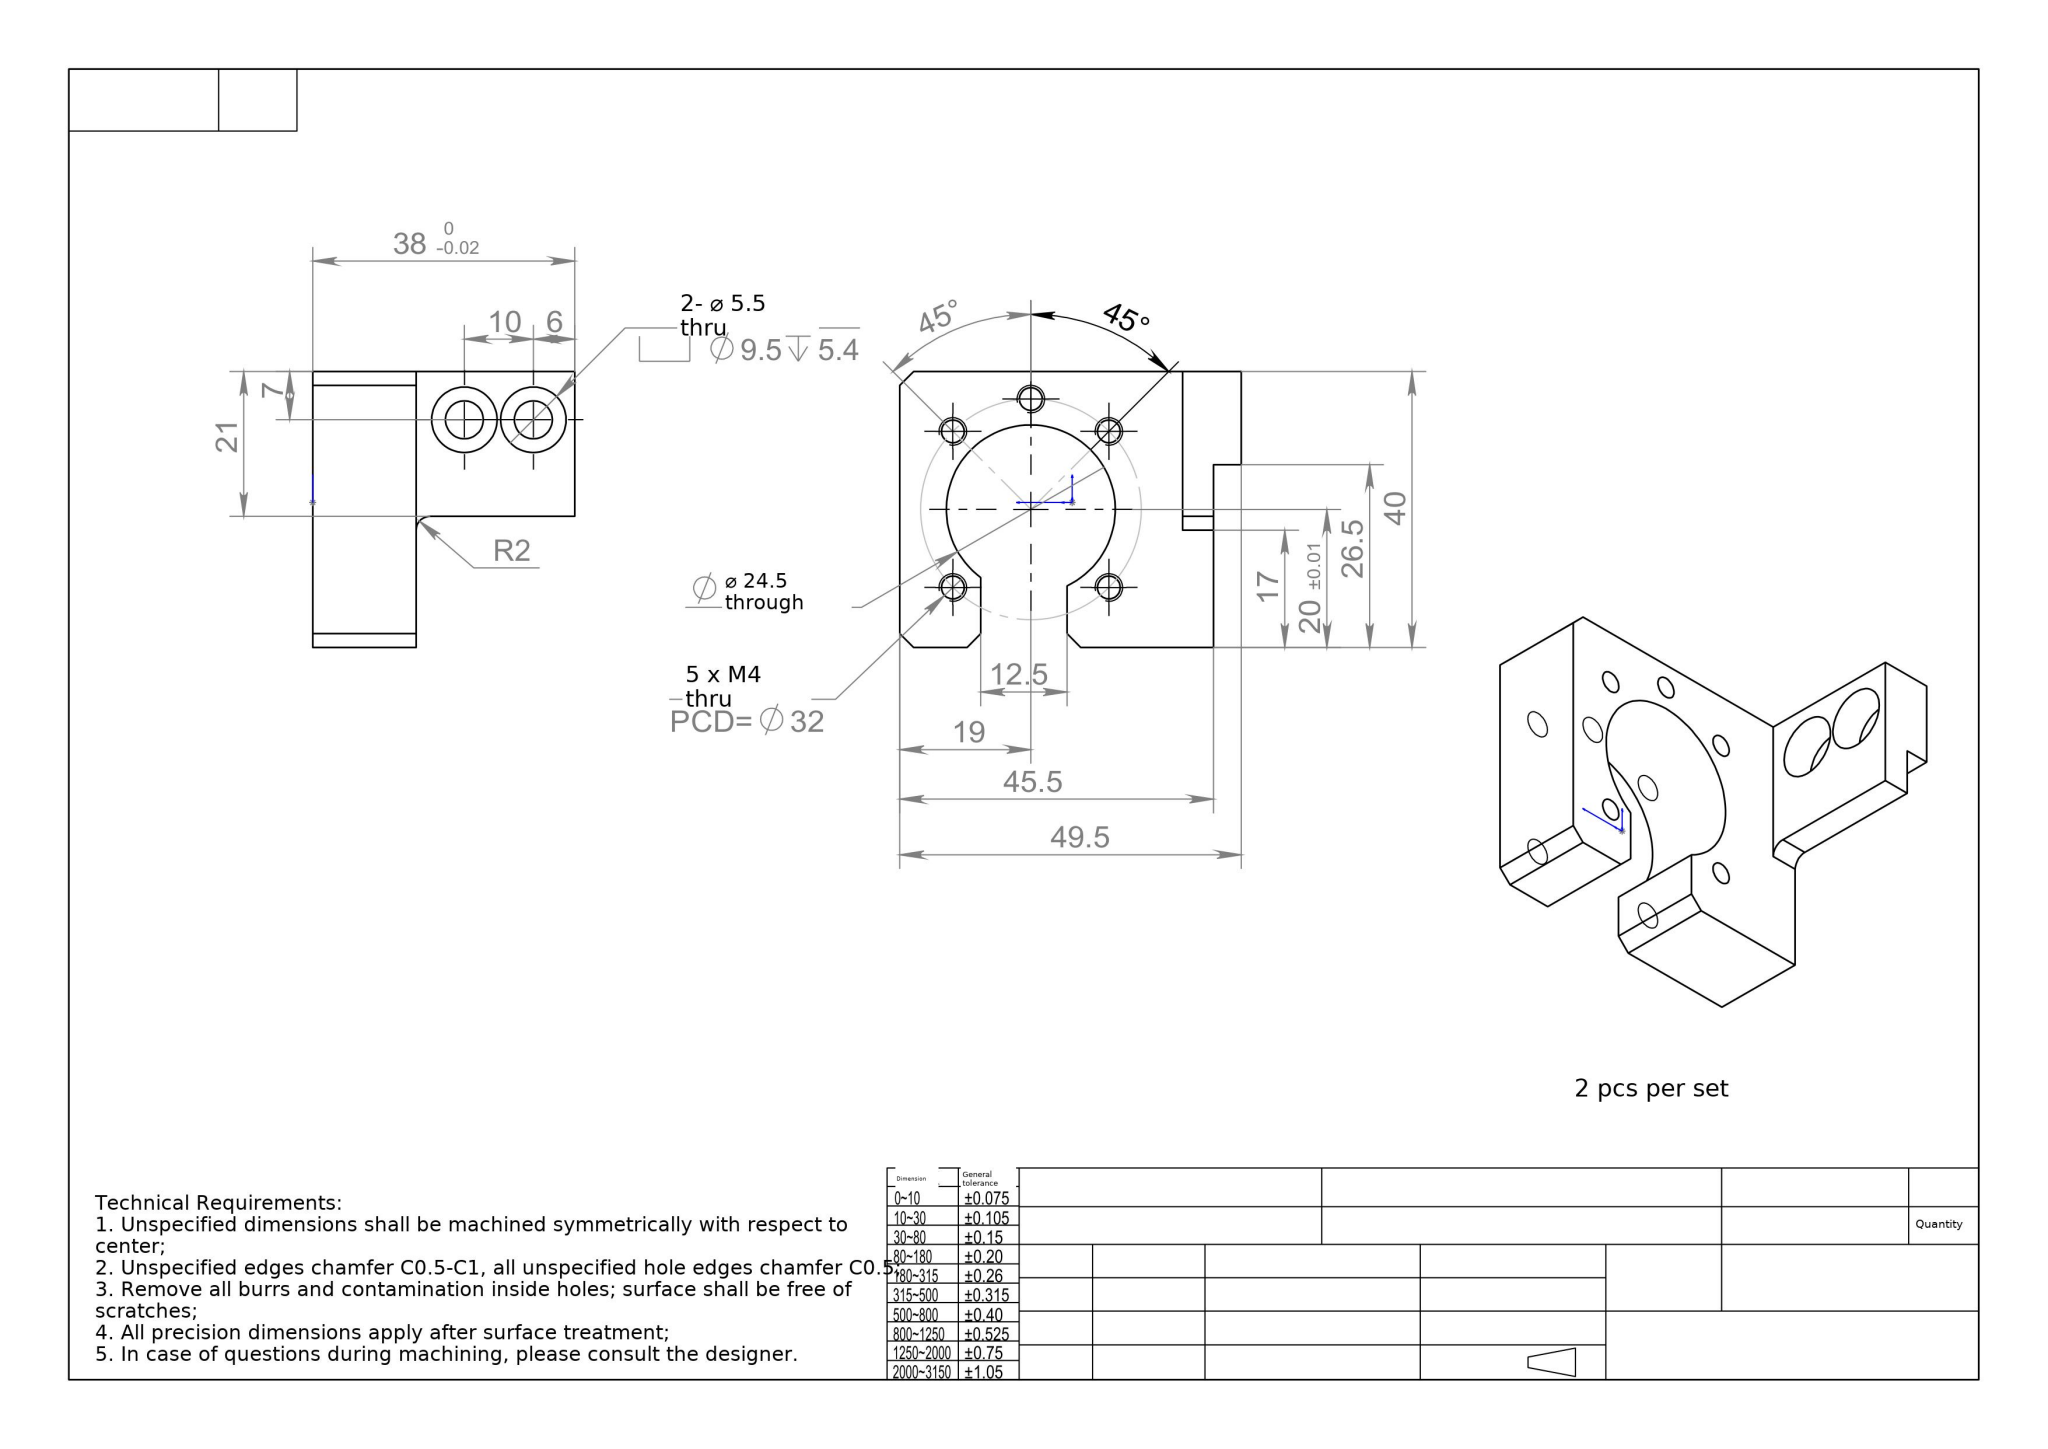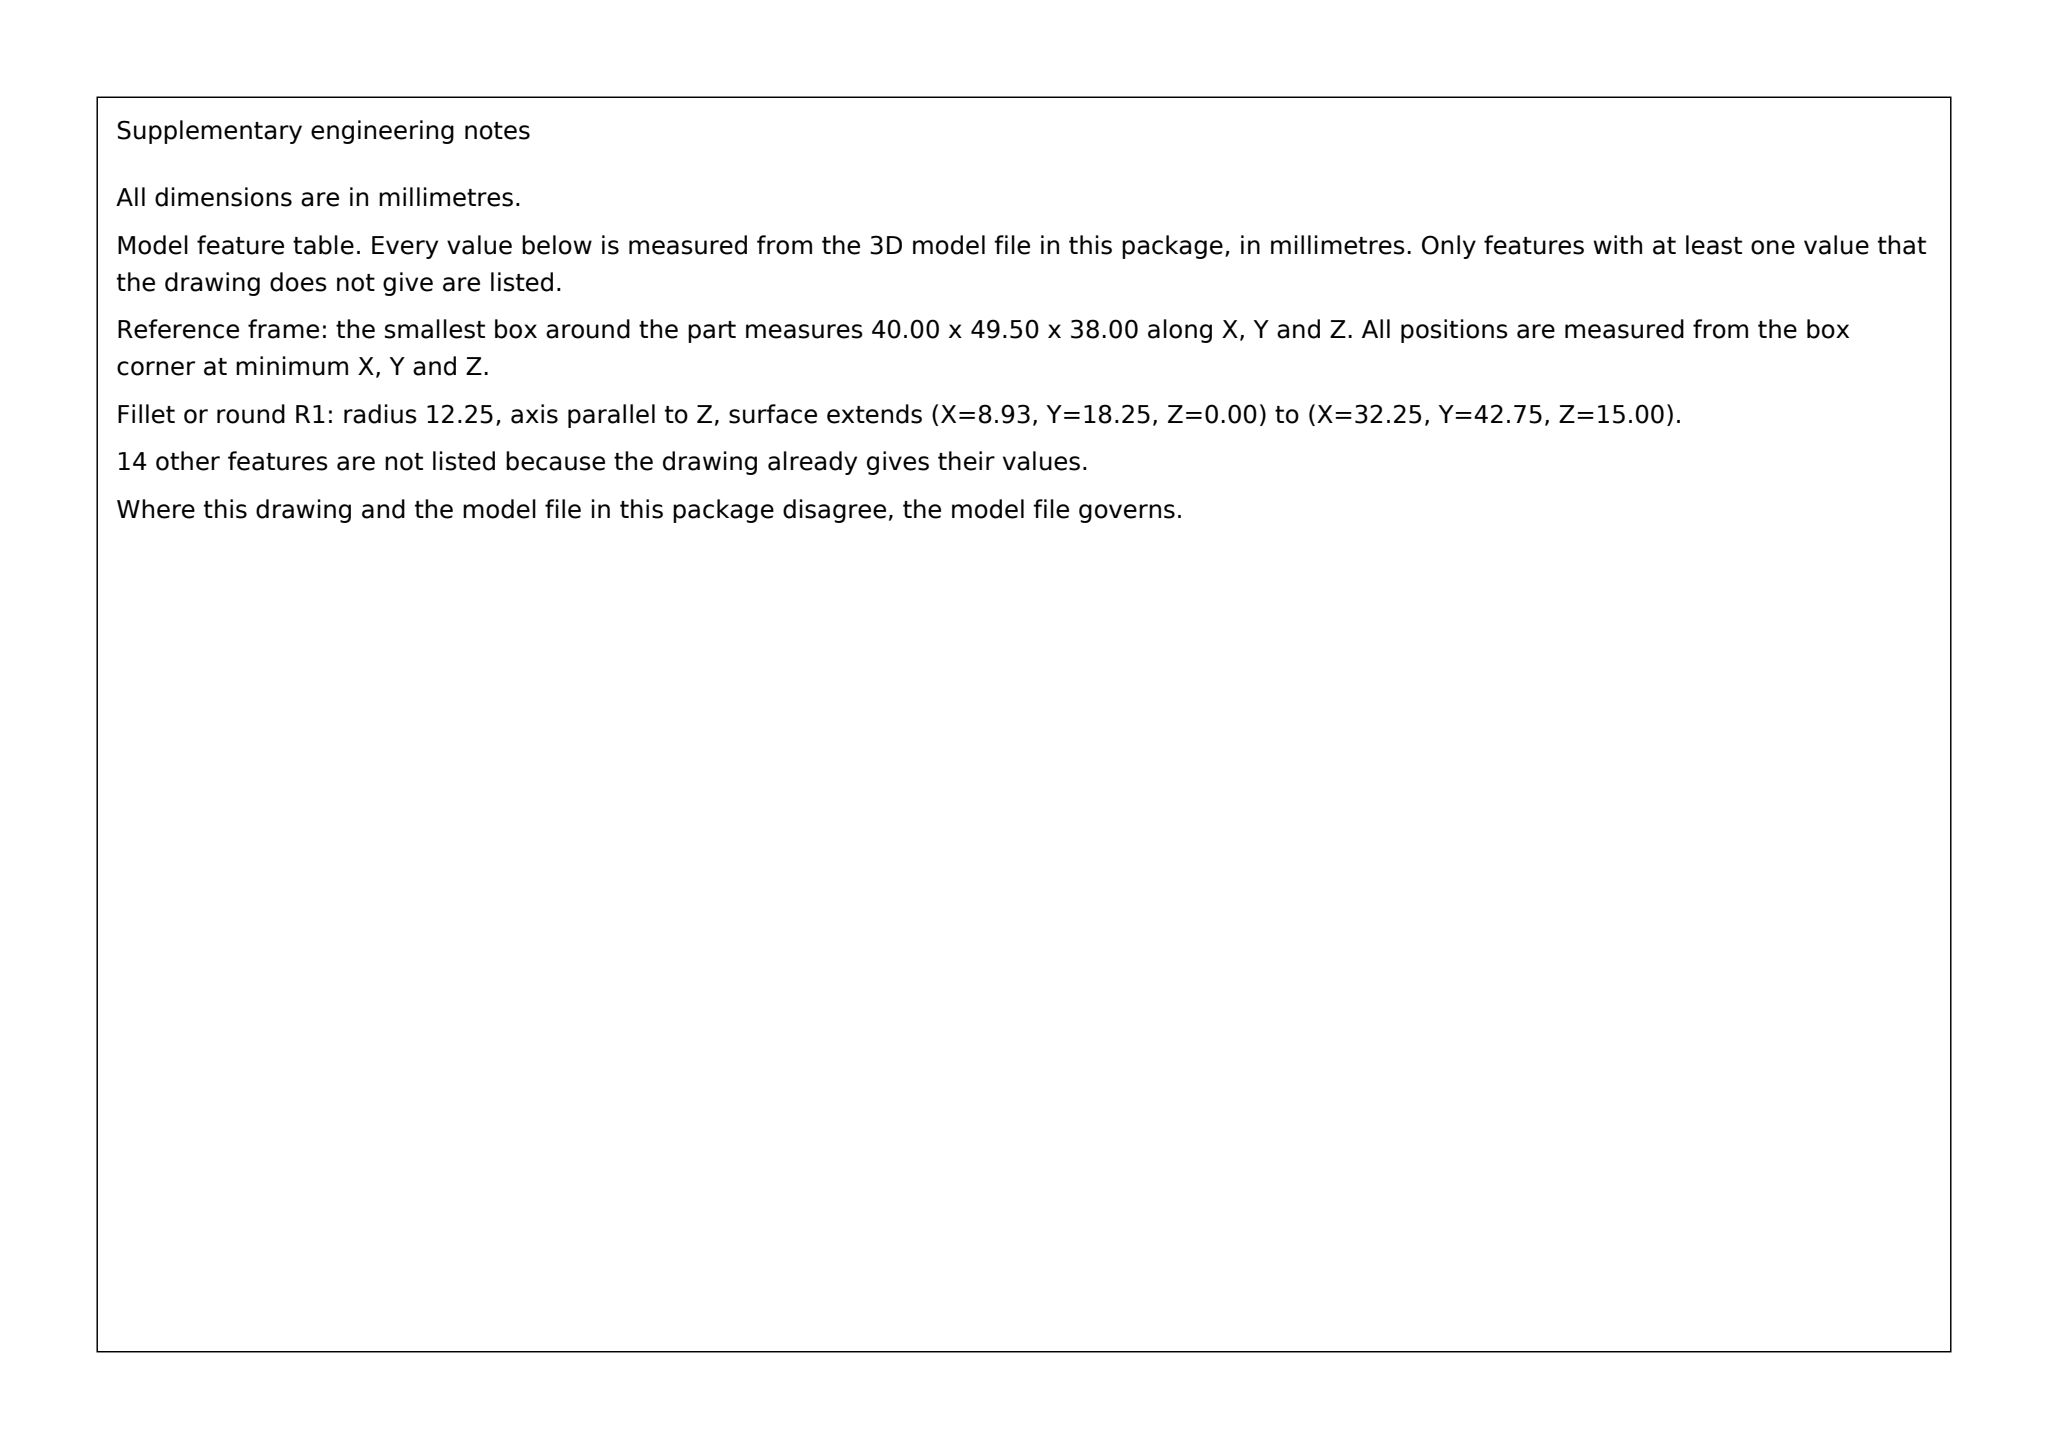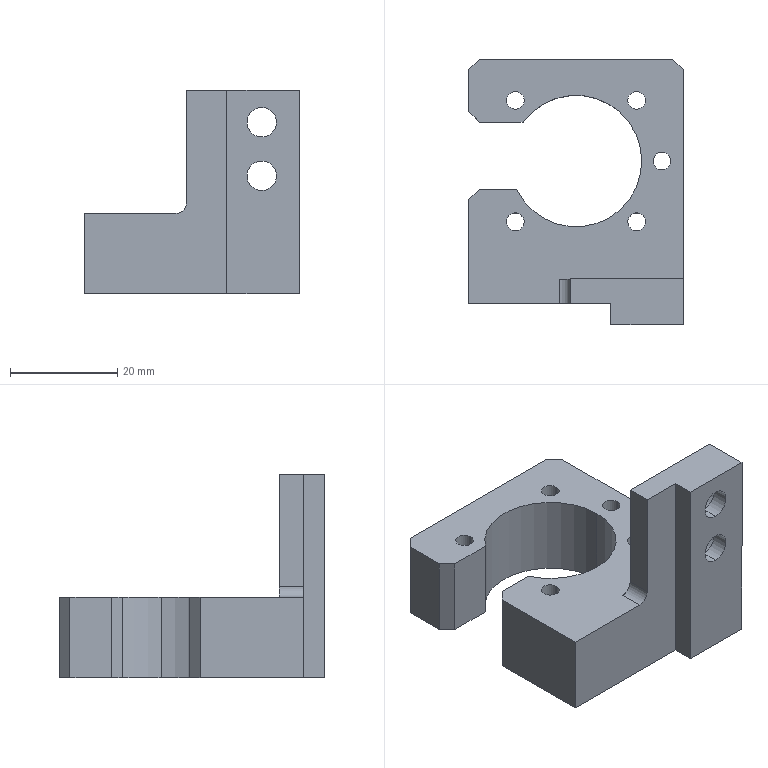Part | SolidWorks | mm | 1 solid | 41 faces | box 40 x 49.5 x 38 mm | volume 21218 mm3 | cylinder 21 | plane 20 | commonest cylinder face diameters 3.3 x10 9.5 x4 5.5 x4 24.5 x2 4 x1
build123d program:
from build123d import *

# Parameters (mm, degrees)
SKETCH1_W                                       = 42
SKETCH1_H                                       = 50
BOSS_EXTRUDE1_DEPTH                             = 15
SKETCH2_W                                       = 23
SKETCH2_H                                       = 9
BOSS_EXTRUDE2_DEPTH                             = 23
FILLET1_R                                       = 2
M5_HEX_SOCKET_HEAD_CAP_SCREW_CBORE1_D           = 5.5
M5_HEX_SOCKET_HEAD_CAP_SCREW_CBORE1_CBORE_D     = 9.5
M5_HEX_SOCKET_HEAD_CAP_SCREW_CBORE1_CBORE_DEPTH = 5.4
SKETCH5_R                                       = 12.25
CUT_EXTRUDE1_DEPTH                              = 40.937
SKETCH6_W                                       = 15
SKETCH6_H                                       = 12.5
CUT_EXTRUDE2_DEPTH                              = 40.937
SKETCH8_W                                       = 30
SKETCH8_H                                       = 0.5
CUT_EXTRUDE4_DEPTH                              = 51.1
CHAMFER2_SIZE                                   = 2
BOSS_EXTRUDE3_START                             = 2
SKETCH12_R                                      = 2.75
BOSS_EXTRUDE3_DEPTH                             = 2
M4_TAPPED_HOLE1_D                               = 3.3
SKETCH24_W                                      = 12
SKETCH24_H                                      = 38
CUT_EXTRUDE5_DEPTH                              = 2.5
M5_HEX_SOCKET_HEAD_CAP_SCREW_CBORE2_D           = 5.5
M5_HEX_SOCKET_HEAD_CAP_SCREW_CBORE2_CBORE_D     = 9.5
M5_HEX_SOCKET_HEAD_CAP_SCREW_CBORE2_CBORE_DEPTH = 5.4
SKETCH27_W                                      = 26.5
SKETCH27_H                                      = 4
CUT_EXTRUDE6_DEPTH                              = 51.1
SKETCH28_W                                      = 2
SKETCH28_H                                      = 38
CUT_EXTRUDE7_DEPTH                              = 66.843
CHAMFER3_SIZE                                   = 2


with BuildPart() as part:
    # Sketch1 → Boss-Extrude1 (new body)
    with BuildSketch(Plane.XY):
        Rectangle(SKETCH1_W, SKETCH1_H)
    extrude(amount=BOSS_EXTRUDE1_DEPTH)

    # Sketch2 → Boss-Extrude2 (add)
    with BuildSketch(Plane.XY.offset(15)):
        with Locations((9.5, -20.5)):
            Rectangle(SKETCH2_W, SKETCH2_H)
    extrude(amount=BOSS_EXTRUDE2_DEPTH)

    # Fillet1
    fillet1_edges = [part.edges().sort_by_distance(p)[0] for p in [
        (-2, -20.5, 15),
    ]]
    fillet(fillet1_edges, radius=FILLET1_R)

    # M5 Hex Socket Head Cap Screw CBORE1 (through all)
    with Locations(Plane(origin=(0, -16, 0), x_dir=(1, 0, 0), z_dir=(0, 1, 0))):
        with Locations((12, -32)):
            CounterBoreHole(M5_HEX_SOCKET_HEAD_CAP_SCREW_CBORE1_D / 2, M5_HEX_SOCKET_HEAD_CAP_SCREW_CBORE1_CBORE_D / 2, M5_HEX_SOCKET_HEAD_CAP_SCREW_CBORE1_CBORE_DEPTH)

    # Sketch5 → Cut-Extrude1 (cut, through all)
    with BuildSketch(Plane.XY.offset(15)):
        with Locations((-1, 6)):
            Circle(SKETCH5_R)
    extrude(amount=-CUT_EXTRUDE1_DEPTH, mode=Mode.SUBTRACT)

    # Sketch6 → Cut-Extrude2 (cut, through all)
    with BuildSketch(Plane.XY.offset(15)):
        with Locations((-13.5, 7)):
            Rectangle(SKETCH6_W, SKETCH6_H)
    extrude(amount=-CUT_EXTRUDE2_DEPTH, mode=Mode.SUBTRACT)

    # Sketch8 → Cut-Extrude4 (cut, through all)
    with BuildSketch(Plane(origin=(0, 0, 0), x_dir=(-1, 0, 0), z_dir=(0, 0, -1))):
        with Locations((6, -24.75)):
            Rectangle(SKETCH8_W, SKETCH8_H)
    extrude(amount=-CUT_EXTRUDE4_DEPTH, mode=Mode.SUBTRACT)

    # Chamfer2
    chamfer2_edges = [part.edges().sort_by_distance(p)[0] for p in [
        (-21, 13.25, 7.5),
        (-21, 0.75, 7.5),
        (-21, -24.5, 7.5),
        (-21, 25, 7.5),
    ]]
    chamfer(chamfer2_edges, length=CHAMFER2_SIZE)

    # Sketch12 → Boss-Extrude3 (add)
    with BuildSketch(Plane.XZ.offset(25).offset(BOSS_EXTRUDE3_START)):
        Polygon((9, 0), (21, 0), (21, 32), (21, 38), (9, 38), align=None)
        with Locations(Location((12, 32, 0), (0, 0, 90))):
            Circle(SKETCH12_R, mode=Mode.SUBTRACT)
        with Locations(Location((14.75, 21.349, 0), (0, 0, 270))):
            Circle(SKETCH12_R, mode=Mode.SUBTRACT)
    extrude(amount=-BOSS_EXTRUDE3_DEPTH)

    # M4 Tapped Hole1 (through all)
    with Locations(Plane(origin=(0, 0, 0), x_dir=(-1, 0, 0), z_dir=(0, 0, -1))):
        with Locations((-15, 6), (-10.314, 17.314), (-10.314, -5.314), (12.314, -5.314), (12.314, 17.314)):
            Hole(M4_TAPPED_HOLE1_D / 2)

    # Sketch24 → Cut-Extrude5 (cut)
    with BuildSketch(Plane.XZ.offset(27)):
        with Locations((15, 19)):
            Rectangle(SKETCH24_W, SKETCH24_H)
    extrude(amount=-CUT_EXTRUDE5_DEPTH, mode=Mode.SUBTRACT)

    # M5 Hex Socket Head Cap Screw CBORE2 (through all)
    with Locations(Plane(origin=(0, -16, 0), x_dir=(1, 0, 0), z_dir=(0, 1, 0))):
        with Locations((12, -22)):
            CounterBoreHole(M5_HEX_SOCKET_HEAD_CAP_SCREW_CBORE2_D / 2, M5_HEX_SOCKET_HEAD_CAP_SCREW_CBORE2_CBORE_D / 2, M5_HEX_SOCKET_HEAD_CAP_SCREW_CBORE2_CBORE_DEPTH)

    # Sketch27 → Cut-Extrude6 (cut, through all)
    with BuildSketch(Plane(origin=(0, 0, 0), x_dir=(-1, 0, 0), z_dir=(0, 0, -1))):
        with Locations((7.75, -22.5)):
            Rectangle(SKETCH27_W, SKETCH27_H)
    extrude(amount=-CUT_EXTRUDE6_DEPTH, mode=Mode.SUBTRACT)

    # Sketch28 → Cut-Extrude7 (cut, through all)
    with BuildSketch(Plane(origin=(0, 25, 0), x_dir=(1, 0, 0), z_dir=(0, 1, 0))):
        with Locations((20, -19)):
            Rectangle(SKETCH28_W, SKETCH28_H)
    extrude(amount=-CUT_EXTRUDE7_DEPTH, mode=Mode.SUBTRACT)

    # Chamfer3
    chamfer3_edges = [part.edges().sort_by_distance(p)[0] for p in [
        (19, 25, 7.5),
    ]]
    chamfer(chamfer3_edges, length=CHAMFER3_SIZE)


solid = part.part